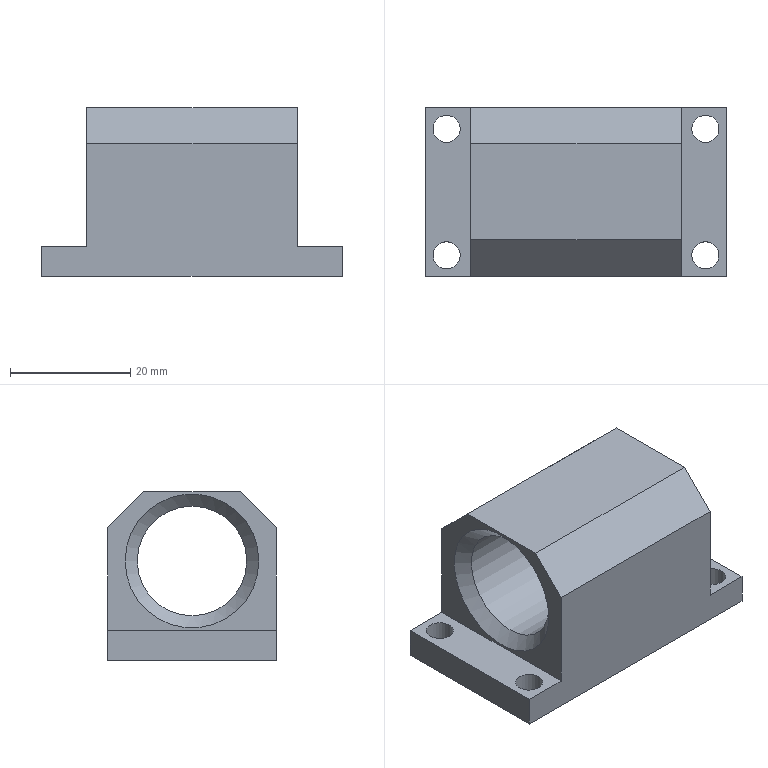Component | NX | WORK_TABLE_NUT | 1 solid | 19 faces | volume 18604 mm3 | plane 12 | cylinder 5 | cone 2 | commonest cylinder face diameters 4.5 x4 18.204 x1